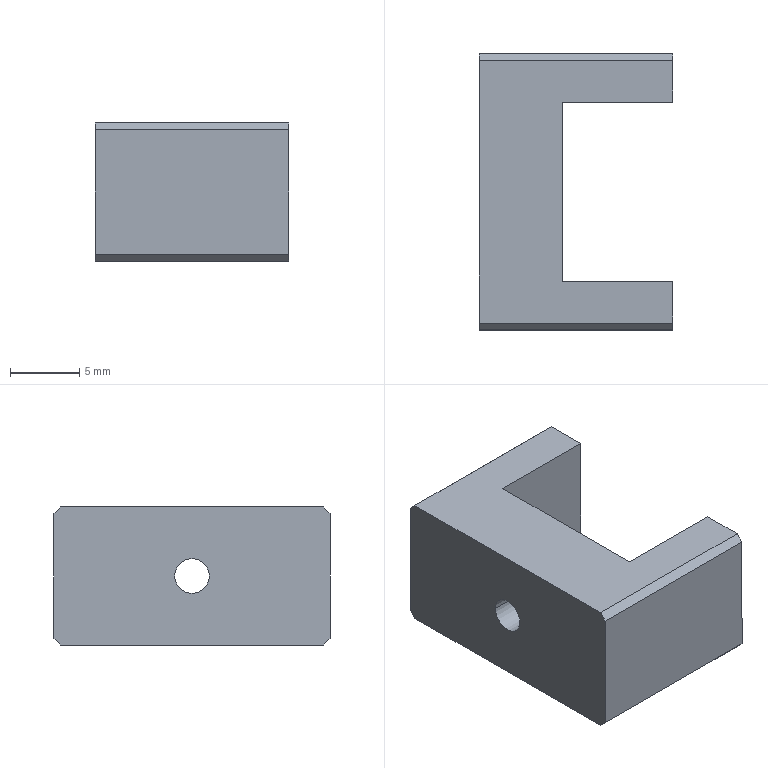Component | SolidWorks | F01AE00111-A2000-21TopEdgeAssembly-1_F01AE00111-A2203-1 | 1 solid | 16 faces | box 14 x 20 x 10 mm | volume 1724 mm3 | plane 14 | cylinder 2 | commonest cylinder face diameters 2.5 x2
build123d program:
from build123d import *

# Parameters (mm, degrees)
SKETCH1_W             = 20
SKETCH1_H             = 10
BOSS_EXTRUDE1_DEPTH   = 14
SKETCH2_W             = 13
SKETCH2_H             = 8
CUT_EXTRUDE1_DEPTH    = 14
CHAMFER1_SIZE         = 0.5
M3_TAPPED_HOLE1_D     = 2.5
M3_TAPPED_HOLE1_DEPTH = 7.5
M3_TAPPED_HOLE1_TIP   = 0.7511


with BuildPart() as part:
    # Sketch1 → Boss-Extrude1 (new body)
    with BuildSketch(Plane.XY):
        with Locations((10, 5)):
            Rectangle(SKETCH1_W, SKETCH1_H)
    extrude(amount=BOSS_EXTRUDE1_DEPTH)

    # Sketch2 → Cut-Extrude1 (cut)
    with BuildSketch(Plane(origin=(0, 10, 0), x_dir=(1, 0, 0), z_dir=(0, 1, 0))):
        with Locations((10, -4)):
            Rectangle(SKETCH2_W, SKETCH2_H)
    extrude(amount=-CUT_EXTRUDE1_DEPTH, mode=Mode.SUBTRACT)

    # Chamfer1
    chamfer1_edges = [part.edges().sort_by_distance(p)[0] for p in [
        (0, 10, 7),
        (20, 10, 7),
        (20, 0, 7),
        (0, 0, 7),
    ]]
    chamfer(chamfer1_edges, length=CHAMFER1_SIZE)

    # M3 Tapped Hole1
    with Locations(Plane.XY.offset(14)):
        with Locations((10, 5)):
            Hole(M3_TAPPED_HOLE1_D / 2, depth=M3_TAPPED_HOLE1_DEPTH)
            with Locations((0, 0, -(M3_TAPPED_HOLE1_DEPTH + M3_TAPPED_HOLE1_TIP / 2))):  # 118° drill point
                Cone(0, M3_TAPPED_HOLE1_D / 2, M3_TAPPED_HOLE1_TIP, mode=Mode.SUBTRACT)


solid = part.part

# Placed as in the assembly
solid = solid.moved(Location((-131.352, 92.298, -37.475), (90, -90, 0)))
STEP:
#1=CARTESIAN_POINT('',(-5.486,3.289,-1.279));
#2=VERTEX_POINT('',#1);
#3=CARTESIAN_POINT('',(-5.486,3.191,-1.279));
#4=VERTEX_POINT('',#3);
#5=CARTESIAN_POINT('',(-5.486,3.24,-1.279));
#6=DIRECTION('',(-1.,-0.,-0.));
#7=DIRECTION('',(0.,-1.,0.));
#8=AXIS2_PLACEMENT_3D('',#5,#6,#7);
#9=CIRCLE('',#8,0.04921);
#10=EDGE_CURVE('',#2,#4,#9,.T.);
#11=ORIENTED_EDGE('',*,*,#10,.F.);
#12=CARTESIAN_POINT('',(-5.723,3.289,-1.279));
#13=VERTEX_POINT('',#12);
#14=CARTESIAN_POINT('',(-5.723,3.289,-1.279));
#15=DIRECTION('',(-1.,-0.,-0.));
#16=VECTOR('',#15,39.37);
#17=LINE('',#14,#16);
#18=EDGE_CURVE('',#2,#13,#17,.T.);
#19=ORIENTED_EDGE('',*,*,#18,.T.);
#20=CARTESIAN_POINT('',(-5.723,3.191,-1.279));
#21=VERTEX_POINT('',#20);
#22=CARTESIAN_POINT('',(-5.723,3.24,-1.279));
#23=DIRECTION('',(-1.,-0.,-0.));
#24=DIRECTION('',(0.,-1.,0.));
#25=AXIS2_PLACEMENT_3D('',#22,#23,#24);
#26=CIRCLE('',#25,0.04921);
#27=EDGE_CURVE('',#13,#21,#26,.T.);
#28=ORIENTED_EDGE('',*,*,#27,.T.);
#29=CARTESIAN_POINT('',(-5.723,3.191,-1.279));
#30=DIRECTION('',(-1.,-0.,-0.));
#31=VECTOR('',#30,39.37);
#32=LINE('',#29,#31);
#33=EDGE_CURVE('',#4,#21,#32,.T.);
#34=ORIENTED_EDGE('',*,*,#33,.F.);
#35=EDGE_LOOP('',(#11,#19,#28,#34));
#36=FACE_OUTER_BOUND('',#35,.T.);
#37=CARTESIAN_POINT('',(-5.723,3.24,-1.279));
#38=DIRECTION('',(-1.,-0.,-0.));
#39=DIRECTION('',(0.,-1.,0.));
#40=AXIS2_PLACEMENT_3D('',#37,#38,#39);
#41=CYLINDRICAL_SURFACE('',#40,0.04921);
#42=ADVANCED_FACE('',(#36),#41,.F.);
#43=CARTESIAN_POINT('',(-5.171,2.866,-1.082));
#44=VERTEX_POINT('',#43);
#45=CARTESIAN_POINT('',(-5.171,2.984,-1.082));
#46=VERTEX_POINT('',#45);
#47=CARTESIAN_POINT('',(-5.171,3.634,-1.082));
#48=DIRECTION('',(-0.,1.,0.));
#49=VECTOR('',#48,39.37);
#50=LINE('',#47,#49);
#51=EDGE_CURVE('',#44,#46,#50,.T.);
#52=ORIENTED_EDGE('',*,*,#51,.F.);
#53=CARTESIAN_POINT('',(-5.171,2.846,-1.101));
#54=VERTEX_POINT('',#53);
#55=CARTESIAN_POINT('',(-5.171,3.053,-0.8947));
#56=DIRECTION('',(0.,-0.7071,-0.7071));
#57=VECTOR('',#56,39.37);
#58=LINE('',#55,#57);
#59=EDGE_CURVE('',#44,#54,#58,.T.);
#60=ORIENTED_EDGE('',*,*,#59,.T.);
#61=CARTESIAN_POINT('',(-5.171,2.846,-1.456));
#62=VERTEX_POINT('',#61);
#63=CARTESIAN_POINT('',(-5.171,2.846,-1.475));
#64=DIRECTION('',(-0.,-0.,1.));
#65=VECTOR('',#64,39.37);
#66=LINE('',#63,#65);
#67=EDGE_CURVE('',#62,#54,#66,.T.);
#68=ORIENTED_EDGE('',*,*,#67,.F.);
#69=CARTESIAN_POINT('',(-5.171,2.866,-1.475));
#70=VERTEX_POINT('',#69);
#71=CARTESIAN_POINT('',(-5.171,3.25,-1.859));
#72=DIRECTION('',(-0.,0.7071,-0.7071));
#73=VECTOR('',#72,39.37);
#74=LINE('',#71,#73);
#75=EDGE_CURVE('',#62,#70,#74,.T.);
#76=ORIENTED_EDGE('',*,*,#75,.T.);
#77=CARTESIAN_POINT('',(-5.171,2.984,-1.475));
#78=VERTEX_POINT('',#77);
#79=CARTESIAN_POINT('',(-5.171,3.634,-1.475));
#80=DIRECTION('',(0.,-1.,-0.));
#81=VECTOR('',#80,39.37);
#82=LINE('',#79,#81);
#83=EDGE_CURVE('',#78,#70,#82,.T.);
#84=ORIENTED_EDGE('',*,*,#83,.F.);
#85=CARTESIAN_POINT('',(-5.171,2.984,-1.475));
#86=DIRECTION('',(0.,0.,-1.));
#87=VECTOR('',#86,39.37);
#88=LINE('',#85,#87);
#89=EDGE_CURVE('',#46,#78,#88,.T.);
#90=ORIENTED_EDGE('',*,*,#89,.F.);
#91=EDGE_LOOP('',(#52,#60,#68,#76,#84,#90));
#92=FACE_OUTER_BOUND('',#91,.T.);
#93=CARTESIAN_POINT('',(-5.171,3.634,-1.475));
#94=DIRECTION('',(1.,0.,0.));
#95=DIRECTION('',(-0.,1.,0.));
#96=AXIS2_PLACEMENT_3D('',#93,#94,#95);
#97=PLANE('',#96);
#98=ADVANCED_FACE('',(#92),#97,.T.);
#99=CARTESIAN_POINT('',(-5.723,3.634,-1.101));
#100=VERTEX_POINT('',#99);
#101=CARTESIAN_POINT('',(-5.723,3.634,-1.456));
#102=VERTEX_POINT('',#101);
#103=CARTESIAN_POINT('',(-5.723,3.634,-1.475));
#104=DIRECTION('',(0.,0.,-1.));
#105=VECTOR('',#104,39.37);
#106=LINE('',#103,#105);
#107=EDGE_CURVE('',#100,#102,#106,.T.);
#108=ORIENTED_EDGE('',*,*,#107,.F.);
#109=CARTESIAN_POINT('',(-5.171,3.634,-1.101));
#110=VERTEX_POINT('',#109);
#111=CARTESIAN_POINT('',(-5.723,3.634,-1.101));
#112=DIRECTION('',(1.,0.,0.));
#113=VECTOR('',#112,39.37);
#114=LINE('',#111,#113);
#115=EDGE_CURVE('',#100,#110,#114,.T.);
#116=ORIENTED_EDGE('',*,*,#115,.T.);
#117=CARTESIAN_POINT('',(-5.171,3.634,-1.456));
#118=VERTEX_POINT('',#117);
#119=CARTESIAN_POINT('',(-5.171,3.634,-1.475));
#120=DIRECTION('',(0.,0.,-1.));
#121=VECTOR('',#120,39.37);
#122=LINE('',#119,#121);
#123=EDGE_CURVE('',#110,#118,#122,.T.);
#124=ORIENTED_EDGE('',*,*,#123,.T.);
#125=CARTESIAN_POINT('',(-5.723,3.634,-1.456));
#126=DIRECTION('',(-1.,-0.,-0.));
#127=VECTOR('',#126,39.37);
#128=LINE('',#125,#127);
#129=EDGE_CURVE('',#118,#102,#128,.T.);
#130=ORIENTED_EDGE('',*,*,#129,.T.);
#131=EDGE_LOOP('',(#108,#116,#124,#130));
#132=FACE_OUTER_BOUND('',#131,.T.);
#133=CARTESIAN_POINT('',(-5.723,3.634,-1.475));
#134=DIRECTION('',(0.,-1.,-0.));
#135=DIRECTION('',(1.,0.,0.));
#136=AXIS2_PLACEMENT_3D('',#133,#134,#135);
#137=PLANE('',#136);
#138=ADVANCED_FACE('',(#132),#137,.F.);
#139=ORIENTED_EDGE('',*,*,#83,.T.);
#140=CARTESIAN_POINT('',(-5.723,2.866,-1.475));
#141=VERTEX_POINT('',#140);
#142=CARTESIAN_POINT('',(-5.723,2.866,-1.475));
#143=DIRECTION('',(-1.,-0.,-0.));
#144=VECTOR('',#143,39.37);
#145=LINE('',#142,#144);
#146=EDGE_CURVE('',#70,#141,#145,.T.);
#147=ORIENTED_EDGE('',*,*,#146,.T.);
#148=CARTESIAN_POINT('',(-5.723,3.614,-1.475));
#149=VERTEX_POINT('',#148);
#150=CARTESIAN_POINT('',(-5.723,3.634,-1.475));
#151=DIRECTION('',(0.,-1.,-0.));
#152=VECTOR('',#151,39.37);
#153=LINE('',#150,#152);
#154=EDGE_CURVE('',#149,#141,#153,.T.);
#155=ORIENTED_EDGE('',*,*,#154,.F.);
#156=CARTESIAN_POINT('',(-5.171,3.614,-1.475));
#157=VERTEX_POINT('',#156);
#158=CARTESIAN_POINT('',(-5.723,3.614,-1.475));
#159=DIRECTION('',(1.,0.,0.));
#160=VECTOR('',#159,39.37);
#161=LINE('',#158,#160);
#162=EDGE_CURVE('',#149,#157,#161,.T.);
#163=ORIENTED_EDGE('',*,*,#162,.T.);
#164=CARTESIAN_POINT('',(-5.171,3.496,-1.475));
#165=VERTEX_POINT('',#164);
#166=CARTESIAN_POINT('',(-5.171,3.634,-1.475));
#167=DIRECTION('',(0.,-1.,-0.));
#168=VECTOR('',#167,39.37);
#169=LINE('',#166,#168);
#170=EDGE_CURVE('',#157,#165,#169,.T.);
#171=ORIENTED_EDGE('',*,*,#170,.T.);
#172=CARTESIAN_POINT('',(-5.486,3.496,-1.475));
#173=VERTEX_POINT('',#172);
#174=CARTESIAN_POINT('',(-5.723,3.496,-1.475));
#175=DIRECTION('',(-1.,-0.,-0.));
#176=VECTOR('',#175,39.37);
#177=LINE('',#174,#176);
#178=EDGE_CURVE('',#165,#173,#177,.T.);
#179=ORIENTED_EDGE('',*,*,#178,.T.);
#180=CARTESIAN_POINT('',(-5.486,2.984,-1.475));
#181=VERTEX_POINT('',#180);
#182=CARTESIAN_POINT('',(-5.486,3.634,-1.475));
#183=DIRECTION('',(0.,-1.,-0.));
#184=VECTOR('',#183,39.37);
#185=LINE('',#182,#184);
#186=EDGE_CURVE('',#173,#181,#185,.T.);
#187=ORIENTED_EDGE('',*,*,#186,.T.);
#188=CARTESIAN_POINT('',(-5.723,2.984,-1.475));
#189=DIRECTION('',(1.,0.,0.));
#190=VECTOR('',#189,39.37);
#191=LINE('',#188,#190);
#192=EDGE_CURVE('',#181,#78,#191,.T.);
#193=ORIENTED_EDGE('',*,*,#192,.T.);
#194=EDGE_LOOP('',(#139,#147,#155,#163,#171,#179,#187,#193));
#195=FACE_OUTER_BOUND('',#194,.T.);
#196=CARTESIAN_POINT('',(-5.723,3.634,-1.475));
#197=DIRECTION('',(-0.,-0.,1.));
#198=DIRECTION('',(-1.,-0.,-0.));
#199=AXIS2_PLACEMENT_3D('',#196,#197,#198);
#200=PLANE('',#199);
#201=ADVANCED_FACE('',(#195),#200,.F.);
#202=ORIENTED_EDGE('',*,*,#67,.T.);
#203=CARTESIAN_POINT('',(-5.723,2.846,-1.101));
#204=VERTEX_POINT('',#203);
#205=CARTESIAN_POINT('',(-5.723,2.846,-1.101));
#206=DIRECTION('',(-1.,-0.,-0.));
#207=VECTOR('',#206,39.37);
#208=LINE('',#205,#207);
#209=EDGE_CURVE('',#54,#204,#208,.T.);
#210=ORIENTED_EDGE('',*,*,#209,.T.);
#211=CARTESIAN_POINT('',(-5.723,2.846,-1.456));
#212=VERTEX_POINT('',#211);
#213=CARTESIAN_POINT('',(-5.723,2.846,-1.475));
#214=DIRECTION('',(-0.,-0.,1.));
#215=VECTOR('',#214,39.37);
#216=LINE('',#213,#215);
#217=EDGE_CURVE('',#212,#204,#216,.T.);
#218=ORIENTED_EDGE('',*,*,#217,.F.);
#219=CARTESIAN_POINT('',(-5.723,2.846,-1.456));
#220=DIRECTION('',(1.,0.,0.));
#221=VECTOR('',#220,39.37);
#222=LINE('',#219,#221);
#223=EDGE_CURVE('',#212,#62,#222,.T.);
#224=ORIENTED_EDGE('',*,*,#223,.T.);
#225=EDGE_LOOP('',(#202,#210,#218,#224));
#226=FACE_OUTER_BOUND('',#225,.T.);
#227=CARTESIAN_POINT('',(-5.723,2.846,-1.475));
#228=DIRECTION('',(-0.,1.,0.));
#229=DIRECTION('',(-1.,-0.,-0.));
#230=AXIS2_PLACEMENT_3D('',#227,#228,#229);
#231=PLANE('',#230);
#232=ADVANCED_FACE('',(#226),#231,.F.);
#233=CARTESIAN_POINT('',(-5.171,3.496,-1.082));
#234=VERTEX_POINT('',#233);
#235=CARTESIAN_POINT('',(-5.171,3.614,-1.082));
#236=VERTEX_POINT('',#235);
#237=CARTESIAN_POINT('',(-5.171,3.634,-1.082));
#238=DIRECTION('',(-0.,1.,0.));
#239=VECTOR('',#238,39.37);
#240=LINE('',#237,#239);
#241=EDGE_CURVE('',#234,#236,#240,.T.);
#242=ORIENTED_EDGE('',*,*,#241,.T.);
#243=CARTESIAN_POINT('',(-5.723,3.614,-1.082));
#244=VERTEX_POINT('',#243);
#245=CARTESIAN_POINT('',(-5.723,3.614,-1.082));
#246=DIRECTION('',(-1.,-0.,-0.));
#247=VECTOR('',#246,39.37);
#248=LINE('',#245,#247);
#249=EDGE_CURVE('',#236,#244,#248,.T.);
#250=ORIENTED_EDGE('',*,*,#249,.T.);
#251=CARTESIAN_POINT('',(-5.723,2.866,-1.082));
#252=VERTEX_POINT('',#251);
#253=CARTESIAN_POINT('',(-5.723,3.634,-1.082));
#254=DIRECTION('',(-0.,1.,0.));
#255=VECTOR('',#254,39.37);
#256=LINE('',#253,#255);
#257=EDGE_CURVE('',#252,#244,#256,.T.);
#258=ORIENTED_EDGE('',*,*,#257,.F.);
#259=CARTESIAN_POINT('',(-5.723,2.866,-1.082));
#260=DIRECTION('',(1.,0.,0.));
#261=VECTOR('',#260,39.37);
#262=LINE('',#259,#261);
#263=EDGE_CURVE('',#252,#44,#262,.T.);
#264=ORIENTED_EDGE('',*,*,#263,.T.);
#265=ORIENTED_EDGE('',*,*,#51,.T.);
#266=CARTESIAN_POINT('',(-5.486,2.984,-1.082));
#267=VERTEX_POINT('',#266);
#268=CARTESIAN_POINT('',(-5.486,2.984,-1.082));
#269=DIRECTION('',(1.,0.,0.));
#270=VECTOR('',#269,39.37);
#271=LINE('',#268,#270);
#272=EDGE_CURVE('',#267,#46,#271,.T.);
#273=ORIENTED_EDGE('',*,*,#272,.F.);
#274=CARTESIAN_POINT('',(-5.486,3.496,-1.082));
#275=VERTEX_POINT('',#274);
#276=CARTESIAN_POINT('',(-5.486,3.496,-1.082));
#277=DIRECTION('',(0.,-1.,-0.));
#278=VECTOR('',#277,39.37);
#279=LINE('',#276,#278);
#280=EDGE_CURVE('',#275,#267,#279,.T.);
#281=ORIENTED_EDGE('',*,*,#280,.F.);
#282=CARTESIAN_POINT('',(-5.486,3.496,-1.082));
#283=DIRECTION('',(-1.,-0.,-0.));
#284=VECTOR('',#283,39.37);
#285=LINE('',#282,#284);
#286=EDGE_CURVE('',#234,#275,#285,.T.);
#287=ORIENTED_EDGE('',*,*,#286,.F.);
#288=EDGE_LOOP('',(#242,#250,#258,#264,#265,#273,#281,#287));
#289=FACE_OUTER_BOUND('',#288,.T.);
#290=CARTESIAN_POINT('',(-5.723,3.634,-1.082));
#291=DIRECTION('',(0.,0.,-1.));
#292=DIRECTION('',(1.,0.,0.));
#293=AXIS2_PLACEMENT_3D('',#290,#291,#292);
#294=PLANE('',#293);
#295=ADVANCED_FACE('',(#289),#294,.F.);
#296=CARTESIAN_POINT('',(-5.723,3.24,-1.279));
#297=DIRECTION('',(-1.,-0.,-0.));
#298=DIRECTION('',(0.,-1.,0.));
#299=AXIS2_PLACEMENT_3D('',#296,#297,#298);
#300=CIRCLE('',#299,0.04921);
#301=EDGE_CURVE('',#21,#13,#300,.T.);
#302=ORIENTED_EDGE('',*,*,#301,.F.);
#303=ORIENTED_EDGE('',*,*,#27,.F.);
#304=EDGE_LOOP('',(#302,#303));
#305=FACE_BOUND('',#304,.T.);
#306=ORIENTED_EDGE('',*,*,#257,.T.);
#307=CARTESIAN_POINT('',(-5.723,3.634,-1.101));
#308=DIRECTION('',(-0.,0.7071,-0.7071));
#309=VECTOR('',#308,39.37);
#310=LINE('',#307,#309);
#311=EDGE_CURVE('',#244,#100,#310,.T.);
#312=ORIENTED_EDGE('',*,*,#311,.T.);
#313=ORIENTED_EDGE('',*,*,#107,.T.);
#314=CARTESIAN_POINT('',(-5.723,3.614,-1.475));
#315=DIRECTION('',(0.,-0.7071,-0.7071));
#316=VECTOR('',#315,39.37);
#317=LINE('',#314,#316);
#318=EDGE_CURVE('',#102,#149,#317,.T.);
#319=ORIENTED_EDGE('',*,*,#318,.T.);
#320=ORIENTED_EDGE('',*,*,#154,.T.);
#321=CARTESIAN_POINT('',(-5.723,2.846,-1.456));
#322=DIRECTION('',(0.,-0.7071,0.7071));
#323=VECTOR('',#322,39.37);
#324=LINE('',#321,#323);
#325=EDGE_CURVE('',#141,#212,#324,.T.);
#326=ORIENTED_EDGE('',*,*,#325,.T.);
#327=ORIENTED_EDGE('',*,*,#217,.T.);
#328=CARTESIAN_POINT('',(-5.723,2.866,-1.082));
#329=DIRECTION('',(-0.,0.7071,0.7071));
#330=VECTOR('',#329,39.37);
#331=LINE('',#328,#330);
#332=EDGE_CURVE('',#204,#252,#331,.T.);
#333=ORIENTED_EDGE('',*,*,#332,.T.);
#334=EDGE_LOOP('',(#306,#312,#313,#319,#320,#326,#327,#333));
#335=FACE_OUTER_BOUND('',#334,.T.);
#336=CARTESIAN_POINT('',(-5.723,3.634,-1.475));
#337=DIRECTION('',(1.,0.,0.));
#338=DIRECTION('',(-0.,1.,0.));
#339=AXIS2_PLACEMENT_3D('',#336,#337,#338);
#340=PLANE('',#339);
#341=ADVANCED_FACE('',(#305,#335),#340,.F.);
#342=ORIENTED_EDGE('',*,*,#123,.F.);
#343=CARTESIAN_POINT('',(-5.171,3.821,-1.288));
#344=DIRECTION('',(0.,-0.7071,0.7071));
#345=VECTOR('',#344,39.37);
#346=LINE('',#343,#345);
#347=EDGE_CURVE('',#110,#236,#346,.T.);
#348=ORIENTED_EDGE('',*,*,#347,.T.);
#349=ORIENTED_EDGE('',*,*,#241,.F.);
#350=CARTESIAN_POINT('',(-5.171,3.496,-1.475));
#351=DIRECTION('',(-0.,-0.,1.));
#352=VECTOR('',#351,39.37);
#353=LINE('',#350,#352);
#354=EDGE_CURVE('',#165,#234,#353,.T.);
#355=ORIENTED_EDGE('',*,*,#354,.F.);
#356=ORIENTED_EDGE('',*,*,#170,.F.);
#357=CARTESIAN_POINT('',(-5.171,3.624,-1.466));
#358=DIRECTION('',(-0.,0.7071,0.7071));
#359=VECTOR('',#358,39.37);
#360=LINE('',#357,#359);
#361=EDGE_CURVE('',#157,#118,#360,.T.);
#362=ORIENTED_EDGE('',*,*,#361,.T.);
#363=EDGE_LOOP('',(#342,#348,#349,#355,#356,#362));
#364=FACE_OUTER_BOUND('',#363,.T.);
#365=CARTESIAN_POINT('',(-5.171,3.634,-1.475));
#366=DIRECTION('',(1.,0.,0.));
#367=DIRECTION('',(-0.,1.,0.));
#368=AXIS2_PLACEMENT_3D('',#365,#366,#367);
#369=PLANE('',#368);
#370=ADVANCED_FACE('',(#364),#369,.T.);
#371=CARTESIAN_POINT('',(-5.486,3.24,-1.279));
#372=DIRECTION('',(-1.,-0.,-0.));
#373=DIRECTION('',(0.,-1.,0.));
#374=AXIS2_PLACEMENT_3D('',#371,#372,#373);
#375=CIRCLE('',#374,0.04921);
#376=EDGE_CURVE('',#4,#2,#375,.T.);
#377=ORIENTED_EDGE('',*,*,#376,.T.);
#378=ORIENTED_EDGE('',*,*,#10,.T.);
#379=EDGE_LOOP('',(#377,#378));
#380=FACE_BOUND('',#379,.T.);
#381=CARTESIAN_POINT('',(-5.486,3.496,-1.633));
#382=DIRECTION('',(-0.,-0.,1.));
#383=VECTOR('',#382,39.37);
#384=LINE('',#381,#383);
#385=EDGE_CURVE('',#173,#275,#384,.T.);
#386=ORIENTED_EDGE('',*,*,#385,.T.);
#387=ORIENTED_EDGE('',*,*,#280,.T.);
#388=CARTESIAN_POINT('',(-5.486,2.984,-1.633));
#389=DIRECTION('',(-0.,-0.,1.));
#390=VECTOR('',#389,39.37);
#391=LINE('',#388,#390);
#392=EDGE_CURVE('',#181,#267,#391,.T.);
#393=ORIENTED_EDGE('',*,*,#392,.F.);
#394=ORIENTED_EDGE('',*,*,#186,.F.);
#395=EDGE_LOOP('',(#386,#387,#393,#394));
#396=FACE_OUTER_BOUND('',#395,.T.);
#397=CARTESIAN_POINT('',(-5.486,3.496,-1.633));
#398=DIRECTION('',(-1.,-0.,-0.));
#399=DIRECTION('',(0.,-1.,-0.));
#400=AXIS2_PLACEMENT_3D('',#397,#398,#399);
#401=PLANE('',#400);
#402=ADVANCED_FACE('',(#380,#396),#401,.F.);
#403=ORIENTED_EDGE('',*,*,#392,.T.);
#404=ORIENTED_EDGE('',*,*,#272,.T.);
#405=ORIENTED_EDGE('',*,*,#89,.T.);
#406=ORIENTED_EDGE('',*,*,#192,.F.);
#407=EDGE_LOOP('',(#403,#404,#405,#406));
#408=FACE_OUTER_BOUND('',#407,.T.);
#409=CARTESIAN_POINT('',(-5.486,2.984,-1.633));
#410=DIRECTION('',(0.,-1.,-0.));
#411=DIRECTION('',(1.,0.,0.));
#412=AXIS2_PLACEMENT_3D('',#409,#410,#411);
#413=PLANE('',#412);
#414=ADVANCED_FACE('',(#408),#413,.F.);
#415=ORIENTED_EDGE('',*,*,#354,.T.);
#416=ORIENTED_EDGE('',*,*,#286,.T.);
#417=ORIENTED_EDGE('',*,*,#385,.F.);
#418=ORIENTED_EDGE('',*,*,#178,.F.);
#419=EDGE_LOOP('',(#415,#416,#417,#418));
#420=FACE_OUTER_BOUND('',#419,.T.);
#421=CARTESIAN_POINT('',(-5.486,3.496,-1.633));
#422=DIRECTION('',(-0.,1.,0.));
#423=DIRECTION('',(-1.,-0.,-0.));
#424=AXIS2_PLACEMENT_3D('',#421,#422,#423);
#425=PLANE('',#424);
#426=ADVANCED_FACE('',(#420),#425,.F.);
#427=ORIENTED_EDGE('',*,*,#311,.F.);
#428=ORIENTED_EDGE('',*,*,#249,.F.);
#429=ORIENTED_EDGE('',*,*,#347,.F.);
#430=ORIENTED_EDGE('',*,*,#115,.F.);
#431=EDGE_LOOP('',(#427,#428,#429,#430));
#432=FACE_OUTER_BOUND('',#431,.T.);
#433=CARTESIAN_POINT('',(-5.723,3.634,-1.101));
#434=DIRECTION('',(0.,-0.7071,-0.7071));
#435=DIRECTION('',(1.,0.,0.));
#436=AXIS2_PLACEMENT_3D('',#433,#434,#435);
#437=PLANE('',#436);
#438=ADVANCED_FACE('',(#432),#437,.F.);
#439=ORIENTED_EDGE('',*,*,#332,.F.);
#440=ORIENTED_EDGE('',*,*,#209,.F.);
#441=ORIENTED_EDGE('',*,*,#59,.F.);
#442=ORIENTED_EDGE('',*,*,#263,.F.);
#443=EDGE_LOOP('',(#439,#440,#441,#442));
#444=FACE_OUTER_BOUND('',#443,.T.);
#445=CARTESIAN_POINT('',(-5.723,2.866,-1.082));
#446=DIRECTION('',(-0.,0.7071,-0.7071));
#447=DIRECTION('',(1.,0.,0.));
#448=AXIS2_PLACEMENT_3D('',#445,#446,#447);
#449=PLANE('',#448);
#450=ADVANCED_FACE('',(#444),#449,.F.);
#451=ORIENTED_EDGE('',*,*,#325,.F.);
#452=ORIENTED_EDGE('',*,*,#146,.F.);
#453=ORIENTED_EDGE('',*,*,#75,.F.);
#454=ORIENTED_EDGE('',*,*,#223,.F.);
#455=EDGE_LOOP('',(#451,#452,#453,#454));
#456=FACE_OUTER_BOUND('',#455,.T.);
#457=CARTESIAN_POINT('',(-5.723,2.846,-1.456));
#458=DIRECTION('',(-0.,0.7071,0.7071));
#459=DIRECTION('',(1.,0.,0.));
#460=AXIS2_PLACEMENT_3D('',#457,#458,#459);
#461=PLANE('',#460);
#462=ADVANCED_FACE('',(#456),#461,.F.);
#463=ORIENTED_EDGE('',*,*,#318,.F.);
#464=ORIENTED_EDGE('',*,*,#129,.F.);
#465=ORIENTED_EDGE('',*,*,#361,.F.);
#466=ORIENTED_EDGE('',*,*,#162,.F.);
#467=EDGE_LOOP('',(#463,#464,#465,#466));
#468=FACE_OUTER_BOUND('',#467,.T.);
#469=CARTESIAN_POINT('',(-5.723,3.614,-1.475));
#470=DIRECTION('',(0.,-0.7071,0.7071));
#471=DIRECTION('',(1.,0.,0.));
#472=AXIS2_PLACEMENT_3D('',#469,#470,#471);
#473=PLANE('',#472);
#474=ADVANCED_FACE('',(#468),#473,.F.);
#475=ORIENTED_EDGE('',*,*,#18,.F.);
#476=ORIENTED_EDGE('',*,*,#376,.F.);
#477=ORIENTED_EDGE('',*,*,#33,.T.);
#478=ORIENTED_EDGE('',*,*,#301,.T.);
#479=EDGE_LOOP('',(#475,#476,#477,#478));
#480=FACE_OUTER_BOUND('',#479,.T.);
#481=CARTESIAN_POINT('',(-5.723,3.24,-1.279));
#482=DIRECTION('',(-1.,-0.,-0.));
#483=DIRECTION('',(0.,-1.,0.));
#484=AXIS2_PLACEMENT_3D('',#481,#482,#483);
#485=CYLINDRICAL_SURFACE('',#484,0.04921);
#486=ADVANCED_FACE('',(#480),#485,.F.);
#487=CLOSED_SHELL('',(#42,#98,#138,#201,#232,#295,#341,#370,#402,#414,#426,#438,#450,#462,#474,#486));
#488=MANIFOLD_SOLID_BREP('',#487);
#489=CARTESIAN_POINT('',(0.,0.,0.));
#490=DIRECTION('',(0.,0.,1.));
#491=DIRECTION('',(1.,0.,0.));
#492=AXIS2_PLACEMENT_3D('',#489,#490,#491);
#493=(LENGTH_UNIT()NAMED_UNIT(*)SI_UNIT($,.METRE.));
#494=LENGTH_MEASURE_WITH_UNIT(LENGTH_MEASURE(0.0254),#493);
#495=DIMENSIONAL_EXPONENTS(1.,0.,0.,0.,0.,0.,0.);
#496=(CONVERSION_BASED_UNIT('',#494)LENGTH_UNIT()NAMED_UNIT(#495));
#497=UNCERTAINTY_MEASURE_WITH_UNIT(LENGTH_MEASURE(0.00001),#496,'','');
#498=(NAMED_UNIT(*)PLANE_ANGLE_UNIT()SI_UNIT($,.RADIAN.));
#499=(NAMED_UNIT(*)SI_UNIT($,.STERADIAN.)SOLID_ANGLE_UNIT());
#500=(GEOMETRIC_REPRESENTATION_CONTEXT(3)GLOBAL_UNCERTAINTY_ASSIGNED_CONTEXT((#497))GLOBAL_UNIT_ASSIGNED_CONTEXT((#496,#498,#499))REPRESENTATION_CONTEXT('',''));
#501=ADVANCED_BREP_SHAPE_REPRESENTATION('',(#488,#492),#500);
#502=COLOUR_RGB('',0.7922,0.8196,0.9333);
#503=FILL_AREA_STYLE_COLOUR('',#502);
#504=FILL_AREA_STYLE('',(#503));
#505=SURFACE_STYLE_FILL_AREA(#504);
#506=SURFACE_SIDE_STYLE('',(#505));
#507=SURFACE_STYLE_USAGE(.BOTH.,#506);
#508=PRESENTATION_STYLE_ASSIGNMENT((#507));
#509=STYLED_ITEM('',(#508),#488);
#510=PRESENTATION_LAYER_ASSIGNMENT('','',(#509));
#511=(LENGTH_UNIT()NAMED_UNIT(*)SI_UNIT($,.METRE.));
#512=LENGTH_MEASURE_WITH_UNIT(LENGTH_MEASURE(0.0254),#511);
#513=DIMENSIONAL_EXPONENTS(1.,0.,0.,0.,0.,0.,0.);
#514=(CONVERSION_BASED_UNIT('',#512)LENGTH_UNIT()NAMED_UNIT(#513));
#515=UNCERTAINTY_MEASURE_WITH_UNIT(LENGTH_MEASURE(0.00001),#514,'','');
#516=(NAMED_UNIT(*)PLANE_ANGLE_UNIT()SI_UNIT($,.RADIAN.));
#517=(NAMED_UNIT(*)SI_UNIT($,.STERADIAN.)SOLID_ANGLE_UNIT());
#518=(GEOMETRIC_REPRESENTATION_CONTEXT(3)GLOBAL_UNCERTAINTY_ASSIGNED_CONTEXT((#515))GLOBAL_UNIT_ASSIGNED_CONTEXT((#514,#516,#517))REPRESENTATION_CONTEXT('',''));
#519=MECHANICAL_DESIGN_GEOMETRIC_PRESENTATION_REPRESENTATION('',(#509),#518);